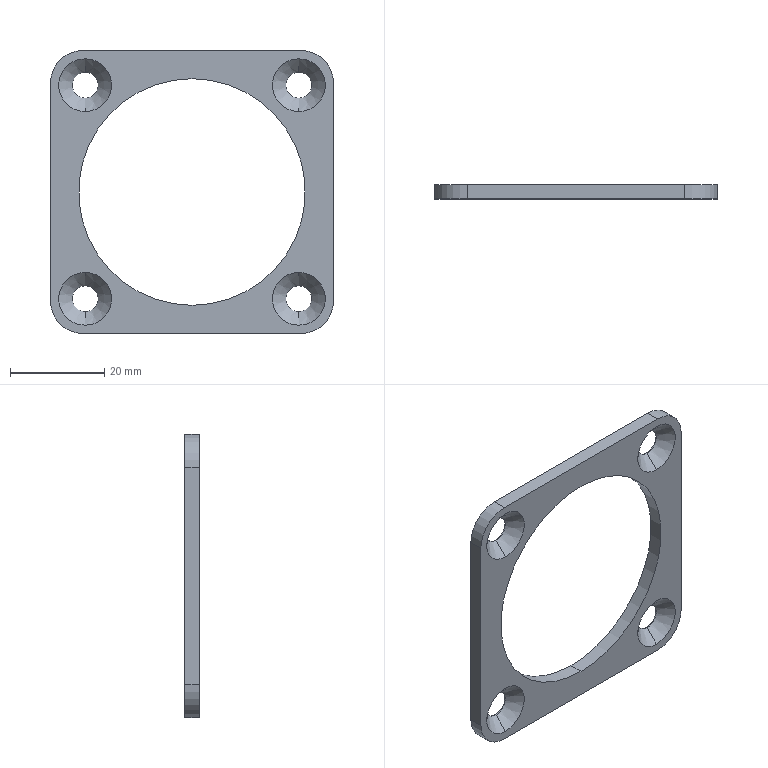Component | SolidWorks | H2020022-0406-1-2 | 1 solid | 28 faces | box 60 x 3 x 60 mm | volume 4582 mm3 | cylinder 14 | cone 8 | plane 6 | commonest cylinder face diameters 5.5 x8 14 x4 48 x2 | material SUS304
build123d program:
from build123d import *

# Parameters (mm, degrees)
SKETCH2_W           = 60
SKETCH2_H           = 60
SKETCH2_R           = 24
BOSS_EXTRUDE1_DEPTH = 3
CIRPATTERN1_COUNT   = 4
FILLET1_R           = 7


with BuildPart() as part:
    # Sketch2 → Boss-Extrude1 (new body)
    with BuildSketch(Plane(origin=(0, 0, 0), x_dir=(1, 0, 0), z_dir=(0, 1, 0))):
        Rectangle(SKETCH2_W, SKETCH2_H)
        with Locations(Location((0, 0, 0), (0, 0, 270))):
            Circle(SKETCH2_R, mode=Mode.SUBTRACT)
    extrude(amount=BOSS_EXTRUDE1_DEPTH)

    # Sketch4 → Countersunk Hole for M5 Hexagon Socket C (revolve, cut)
    with BuildSketch(Plane(origin=(-22.627, 3, -22.627), x_dir=(0, 0, 1), z_dir=(1, 0, 0))):
        Polygon((0, 0), (0, 3), (2.75, 3), (2.75, 2.85), (5.6, 0), align=None)
    countersunk_hole_for_m5_hexagon_socket_c = revolve(axis=Axis((-22.627, 9.35, -22.627), (0, -1, 0)), mode=Mode.SUBTRACT)

    # CirPattern1: Countersunk Hole for M5 Hexagon Socket C ×4 about axis
    cirpattern1_axis = Axis((0, 0, 0), (0, 1, 0))
    for i in range(1, CIRPATTERN1_COUNT):
        add(countersunk_hole_for_m5_hexagon_socket_c.rotate(cirpattern1_axis, i * 360 / CIRPATTERN1_COUNT), mode=Mode.SUBTRACT)

    # Fillet1
    fillet1_edges = [part.edges().sort_by_distance(p)[0] for p in [
        (30, 1.5, 30),
        (-30, 1.5, 30),
        (-30, 1.5, -30),
        (30, 1.5, -30),
    ]]
    fillet(fillet1_edges, radius=FILLET1_R)


solid = part.part

# Placed as in the assembly
solid = solid.moved(Location((-30.964, 101.813, 280.197), (180, 0, 0)))
STEP:
#1=COLOUR_RGB('',0.7922,0.8196,0.9333);
#2=FILL_AREA_STYLE_COLOUR('',#1);
#3=FILL_AREA_STYLE('',(#2));
#4=SURFACE_STYLE_FILL_AREA(#3);
#5=SURFACE_SIDE_STYLE('',(#4));
#6=SURFACE_STYLE_USAGE(.BOTH.,#5);
#7=PRESENTATION_STYLE_ASSIGNMENT((#6));
#8=CARTESIAN_POINT('',(-2.11,4.002,10.032));
#9=VERTEX_POINT('',#8);
#10=CARTESIAN_POINT('',(-2.11,4.002,10.249));
#11=VERTEX_POINT('',#10);
#12=CARTESIAN_POINT('',(-2.11,4.002,10.141));
#13=DIRECTION('',(0.,-1.,0.));
#14=DIRECTION('',(0.,0.,1.));
#15=AXIS2_PLACEMENT_3D('',#12,#13,#14);
#16=CIRCLE('',#15,0.1083);
#17=EDGE_CURVE('',#9,#11,#16,.T.);
#18=ORIENTED_EDGE('',*,*,#17,.F.);
#19=CARTESIAN_POINT('',(-2.11,3.89,9.92));
#20=VERTEX_POINT('',#19);
#21=CARTESIAN_POINT('',(-2.11,3.89,9.92));
#22=DIRECTION('',(-0.,-0.7071,-0.7071));
#23=VECTOR('',#22,39.37);
#24=LINE('',#21,#23);
#25=EDGE_CURVE('',#9,#20,#24,.T.);
#26=ORIENTED_EDGE('',*,*,#25,.T.);
#27=CARTESIAN_POINT('',(-2.11,3.89,10.361));
#28=VERTEX_POINT('',#27);
#29=CARTESIAN_POINT('',(-2.11,3.89,10.141));
#30=DIRECTION('',(0.,-1.,0.));
#31=DIRECTION('',(0.,0.,1.));
#32=AXIS2_PLACEMENT_3D('',#29,#30,#31);
#33=CIRCLE('',#32,0.2205);
#34=EDGE_CURVE('',#20,#28,#33,.T.);
#35=ORIENTED_EDGE('',*,*,#34,.T.);
#36=CARTESIAN_POINT('',(-2.11,3.89,10.361));
#37=DIRECTION('',(0.,-0.7071,0.7071));
#38=VECTOR('',#37,39.37);
#39=LINE('',#36,#38);
#40=EDGE_CURVE('',#11,#28,#39,.T.);
#41=ORIENTED_EDGE('',*,*,#40,.F.);
#42=EDGE_LOOP('',(#18,#26,#35,#41));
#43=FACE_OUTER_BOUND('',#42,.T.);
#44=CARTESIAN_POINT('',(-2.11,3.89,10.141));
#45=DIRECTION('',(0.,-1.,0.));
#46=DIRECTION('',(0.,0.,1.));
#47=AXIS2_PLACEMENT_3D('',#44,#45,#46);
#48=CONICAL_SURFACE('',#47,0.2205,0.7854);
#49=ADVANCED_FACE('',(#43),#48,.F.);
#50=CARTESIAN_POINT('',(-2.11,4.008,10.032));
#51=VERTEX_POINT('',#50);
#52=CARTESIAN_POINT('',(-2.11,4.008,10.249));
#53=VERTEX_POINT('',#52);
#54=CARTESIAN_POINT('',(-2.11,4.008,10.141));
#55=DIRECTION('',(0.,-1.,0.));
#56=DIRECTION('',(0.,0.,1.));
#57=AXIS2_PLACEMENT_3D('',#54,#55,#56);
#58=CIRCLE('',#57,0.1083);
#59=EDGE_CURVE('',#51,#53,#58,.T.);
#60=ORIENTED_EDGE('',*,*,#59,.F.);
#61=CARTESIAN_POINT('',(-2.11,3.89,10.032));
#62=DIRECTION('',(0.,-1.,0.));
#63=VECTOR('',#62,39.37);
#64=LINE('',#61,#63);
#65=EDGE_CURVE('',#51,#9,#64,.T.);
#66=ORIENTED_EDGE('',*,*,#65,.T.);
#67=ORIENTED_EDGE('',*,*,#17,.T.);
#68=CARTESIAN_POINT('',(-2.11,3.89,10.249));
#69=DIRECTION('',(0.,-1.,0.));
#70=VECTOR('',#69,39.37);
#71=LINE('',#68,#70);
#72=EDGE_CURVE('',#53,#11,#71,.T.);
#73=ORIENTED_EDGE('',*,*,#72,.F.);
#74=EDGE_LOOP('',(#60,#66,#67,#73));
#75=FACE_OUTER_BOUND('',#74,.T.);
#76=CARTESIAN_POINT('',(-2.11,3.89,10.141));
#77=DIRECTION('',(0.,-1.,0.));
#78=DIRECTION('',(0.,0.,1.));
#79=AXIS2_PLACEMENT_3D('',#76,#77,#78);
#80=CYLINDRICAL_SURFACE('',#79,0.1083);
#81=ADVANCED_FACE('',(#75),#80,.F.);
#82=CARTESIAN_POINT('',(-2.11,4.002,11.814));
#83=VERTEX_POINT('',#82);
#84=CARTESIAN_POINT('',(-2.11,4.002,12.03));
#85=VERTEX_POINT('',#84);
#86=CARTESIAN_POINT('',(-2.11,4.002,11.922));
#87=DIRECTION('',(0.,-1.,0.));
#88=DIRECTION('',(0.,0.,1.));
#89=AXIS2_PLACEMENT_3D('',#86,#87,#88);
#90=CIRCLE('',#89,0.1083);
#91=EDGE_CURVE('',#83,#85,#90,.T.);
#92=ORIENTED_EDGE('',*,*,#91,.F.);
#93=CARTESIAN_POINT('',(-2.11,3.89,11.702));
#94=VERTEX_POINT('',#93);
#95=CARTESIAN_POINT('',(-2.11,3.89,11.702));
#96=DIRECTION('',(-0.,-0.7071,-0.7071));
#97=VECTOR('',#96,39.37);
#98=LINE('',#95,#97);
#99=EDGE_CURVE('',#83,#94,#98,.T.);
#100=ORIENTED_EDGE('',*,*,#99,.T.);
#101=CARTESIAN_POINT('',(-2.11,3.89,12.143));
#102=VERTEX_POINT('',#101);
#103=CARTESIAN_POINT('',(-2.11,3.89,11.922));
#104=DIRECTION('',(0.,-1.,0.));
#105=DIRECTION('',(0.,0.,1.));
#106=AXIS2_PLACEMENT_3D('',#103,#104,#105);
#107=CIRCLE('',#106,0.2205);
#108=EDGE_CURVE('',#94,#102,#107,.T.);
#109=ORIENTED_EDGE('',*,*,#108,.T.);
#110=CARTESIAN_POINT('',(-2.11,3.89,12.143));
#111=DIRECTION('',(0.,-0.7071,0.7071));
#112=VECTOR('',#111,39.37);
#113=LINE('',#110,#112);
#114=EDGE_CURVE('',#85,#102,#113,.T.);
#115=ORIENTED_EDGE('',*,*,#114,.F.);
#116=EDGE_LOOP('',(#92,#100,#109,#115));
#117=FACE_OUTER_BOUND('',#116,.T.);
#118=CARTESIAN_POINT('',(-2.11,3.89,11.922));
#119=DIRECTION('',(0.,-1.,0.));
#120=DIRECTION('',(0.,0.,1.));
#121=AXIS2_PLACEMENT_3D('',#118,#119,#120);
#122=CONICAL_SURFACE('',#121,0.2205,0.7854);
#123=ADVANCED_FACE('',(#117),#122,.F.);
#124=CARTESIAN_POINT('',(-2.11,4.008,11.814));
#125=VERTEX_POINT('',#124);
#126=CARTESIAN_POINT('',(-2.11,4.008,12.03));
#127=VERTEX_POINT('',#126);
#128=CARTESIAN_POINT('',(-2.11,4.008,11.922));
#129=DIRECTION('',(0.,-1.,0.));
#130=DIRECTION('',(0.,0.,1.));
#131=AXIS2_PLACEMENT_3D('',#128,#129,#130);
#132=CIRCLE('',#131,0.1083);
#133=EDGE_CURVE('',#125,#127,#132,.T.);
#134=ORIENTED_EDGE('',*,*,#133,.F.);
#135=CARTESIAN_POINT('',(-2.11,3.89,11.814));
#136=DIRECTION('',(0.,-1.,0.));
#137=VECTOR('',#136,39.37);
#138=LINE('',#135,#137);
#139=EDGE_CURVE('',#125,#83,#138,.T.);
#140=ORIENTED_EDGE('',*,*,#139,.T.);
#141=ORIENTED_EDGE('',*,*,#91,.T.);
#142=CARTESIAN_POINT('',(-2.11,3.89,12.03));
#143=DIRECTION('',(0.,-1.,0.));
#144=VECTOR('',#143,39.37);
#145=LINE('',#142,#144);
#146=EDGE_CURVE('',#127,#85,#145,.T.);
#147=ORIENTED_EDGE('',*,*,#146,.F.);
#148=EDGE_LOOP('',(#134,#140,#141,#147));
#149=FACE_OUTER_BOUND('',#148,.T.);
#150=CARTESIAN_POINT('',(-2.11,3.89,11.922));
#151=DIRECTION('',(0.,-1.,0.));
#152=DIRECTION('',(0.,0.,1.));
#153=AXIS2_PLACEMENT_3D('',#150,#151,#152);
#154=CYLINDRICAL_SURFACE('',#153,0.1083);
#155=ADVANCED_FACE('',(#149),#154,.F.);
#156=CARTESIAN_POINT('',(-0.3282,4.002,11.814));
#157=VERTEX_POINT('',#156);
#158=CARTESIAN_POINT('',(-0.3282,4.002,12.03));
#159=VERTEX_POINT('',#158);
#160=CARTESIAN_POINT('',(-0.3282,4.002,11.922));
#161=DIRECTION('',(0.,-1.,0.));
#162=DIRECTION('',(0.,0.,1.));
#163=AXIS2_PLACEMENT_3D('',#160,#161,#162);
#164=CIRCLE('',#163,0.1083);
#165=EDGE_CURVE('',#157,#159,#164,.T.);
#166=ORIENTED_EDGE('',*,*,#165,.F.);
#167=CARTESIAN_POINT('',(-0.3282,3.89,11.702));
#168=VERTEX_POINT('',#167);
#169=CARTESIAN_POINT('',(-0.3282,3.89,11.702));
#170=DIRECTION('',(-0.,-0.7071,-0.7071));
#171=VECTOR('',#170,39.37);
#172=LINE('',#169,#171);
#173=EDGE_CURVE('',#157,#168,#172,.T.);
#174=ORIENTED_EDGE('',*,*,#173,.T.);
#175=CARTESIAN_POINT('',(-0.3282,3.89,12.143));
#176=VERTEX_POINT('',#175);
#177=CARTESIAN_POINT('',(-0.3282,3.89,11.922));
#178=DIRECTION('',(0.,-1.,0.));
#179=DIRECTION('',(0.,0.,1.));
#180=AXIS2_PLACEMENT_3D('',#177,#178,#179);
#181=CIRCLE('',#180,0.2205);
#182=EDGE_CURVE('',#168,#176,#181,.T.);
#183=ORIENTED_EDGE('',*,*,#182,.T.);
#184=CARTESIAN_POINT('',(-0.3282,3.89,12.143));
#185=DIRECTION('',(0.,-0.7071,0.7071));
#186=VECTOR('',#185,39.37);
#187=LINE('',#184,#186);
#188=EDGE_CURVE('',#159,#176,#187,.T.);
#189=ORIENTED_EDGE('',*,*,#188,.F.);
#190=EDGE_LOOP('',(#166,#174,#183,#189));
#191=FACE_OUTER_BOUND('',#190,.T.);
#192=CARTESIAN_POINT('',(-0.3282,3.89,11.922));
#193=DIRECTION('',(0.,-1.,0.));
#194=DIRECTION('',(0.,0.,1.));
#195=AXIS2_PLACEMENT_3D('',#192,#193,#194);
#196=CONICAL_SURFACE('',#195,0.2205,0.7854);
#197=ADVANCED_FACE('',(#191),#196,.F.);
#198=CARTESIAN_POINT('',(-0.3282,4.008,11.814));
#199=VERTEX_POINT('',#198);
#200=CARTESIAN_POINT('',(-0.3282,4.008,12.03));
#201=VERTEX_POINT('',#200);
#202=CARTESIAN_POINT('',(-0.3282,4.008,11.922));
#203=DIRECTION('',(0.,-1.,0.));
#204=DIRECTION('',(0.,0.,1.));
#205=AXIS2_PLACEMENT_3D('',#202,#203,#204);
#206=CIRCLE('',#205,0.1083);
#207=EDGE_CURVE('',#199,#201,#206,.T.);
#208=ORIENTED_EDGE('',*,*,#207,.F.);
#209=CARTESIAN_POINT('',(-0.3282,3.89,11.814));
#210=DIRECTION('',(0.,-1.,0.));
#211=VECTOR('',#210,39.37);
#212=LINE('',#209,#211);
#213=EDGE_CURVE('',#199,#157,#212,.T.);
#214=ORIENTED_EDGE('',*,*,#213,.T.);
#215=ORIENTED_EDGE('',*,*,#165,.T.);
#216=CARTESIAN_POINT('',(-0.3282,3.89,12.03));
#217=DIRECTION('',(0.,-1.,0.));
#218=VECTOR('',#217,39.37);
#219=LINE('',#216,#218);
#220=EDGE_CURVE('',#201,#159,#219,.T.);
#221=ORIENTED_EDGE('',*,*,#220,.F.);
#222=EDGE_LOOP('',(#208,#214,#215,#221));
#223=FACE_OUTER_BOUND('',#222,.T.);
#224=CARTESIAN_POINT('',(-0.3282,3.89,11.922));
#225=DIRECTION('',(0.,-1.,0.));
#226=DIRECTION('',(0.,0.,1.));
#227=AXIS2_PLACEMENT_3D('',#224,#225,#226);
#228=CYLINDRICAL_SURFACE('',#227,0.1083);
#229=ADVANCED_FACE('',(#223),#228,.F.);
#230=CARTESIAN_POINT('',(-0.3282,4.002,10.032));
#231=VERTEX_POINT('',#230);
#232=CARTESIAN_POINT('',(-0.3282,4.002,10.249));
#233=VERTEX_POINT('',#232);
#234=CARTESIAN_POINT('',(-0.3282,4.002,10.141));
#235=DIRECTION('',(0.,-1.,0.));
#236=DIRECTION('',(0.,0.,1.));
#237=AXIS2_PLACEMENT_3D('',#234,#235,#236);
#238=CIRCLE('',#237,0.1083);
#239=EDGE_CURVE('',#231,#233,#238,.T.);
#240=ORIENTED_EDGE('',*,*,#239,.F.);
#241=CARTESIAN_POINT('',(-0.3282,3.89,9.92));
#242=VERTEX_POINT('',#241);
#243=CARTESIAN_POINT('',(-0.3282,3.89,9.92));
#244=DIRECTION('',(-0.,-0.7071,-0.7071));
#245=VECTOR('',#244,39.37);
#246=LINE('',#243,#245);
#247=EDGE_CURVE('',#231,#242,#246,.T.);
#248=ORIENTED_EDGE('',*,*,#247,.T.);
#249=CARTESIAN_POINT('',(-0.3282,3.89,10.361));
#250=VERTEX_POINT('',#249);
#251=CARTESIAN_POINT('',(-0.3282,3.89,10.141));
#252=DIRECTION('',(0.,-1.,0.));
#253=DIRECTION('',(0.,0.,1.));
#254=AXIS2_PLACEMENT_3D('',#251,#252,#253);
#255=CIRCLE('',#254,0.2205);
#256=EDGE_CURVE('',#242,#250,#255,.T.);
#257=ORIENTED_EDGE('',*,*,#256,.T.);
#258=CARTESIAN_POINT('',(-0.3282,3.89,10.361));
#259=DIRECTION('',(0.,-0.7071,0.7071));
#260=VECTOR('',#259,39.37);
#261=LINE('',#258,#260);
#262=EDGE_CURVE('',#233,#250,#261,.T.);
#263=ORIENTED_EDGE('',*,*,#262,.F.);
#264=EDGE_LOOP('',(#240,#248,#257,#263));
#265=FACE_OUTER_BOUND('',#264,.T.);
#266=CARTESIAN_POINT('',(-0.3282,3.89,10.141));
#267=DIRECTION('',(0.,-1.,0.));
#268=DIRECTION('',(0.,0.,1.));
#269=AXIS2_PLACEMENT_3D('',#266,#267,#268);
#270=CONICAL_SURFACE('',#269,0.2205,0.7854);
#271=ADVANCED_FACE('',(#265),#270,.F.);
#272=CARTESIAN_POINT('',(-0.3282,4.008,10.032));
#273=VERTEX_POINT('',#272);
#274=CARTESIAN_POINT('',(-0.3282,4.008,10.249));
#275=VERTEX_POINT('',#274);
#276=CARTESIAN_POINT('',(-0.3282,4.008,10.141));
#277=DIRECTION('',(0.,-1.,0.));
#278=DIRECTION('',(0.,0.,1.));
#279=AXIS2_PLACEMENT_3D('',#276,#277,#278);
#280=CIRCLE('',#279,0.1083);
#281=EDGE_CURVE('',#273,#275,#280,.T.);
#282=ORIENTED_EDGE('',*,*,#281,.F.);
#283=CARTESIAN_POINT('',(-0.3282,3.89,10.032));
#284=DIRECTION('',(0.,-1.,0.));
#285=VECTOR('',#284,39.37);
#286=LINE('',#283,#285);
#287=EDGE_CURVE('',#273,#231,#286,.T.);
#288=ORIENTED_EDGE('',*,*,#287,.T.);
#289=ORIENTED_EDGE('',*,*,#239,.T.);
#290=CARTESIAN_POINT('',(-0.3282,3.89,10.249));
#291=DIRECTION('',(0.,-1.,0.));
#292=VECTOR('',#291,39.37);
#293=LINE('',#290,#292);
#294=EDGE_CURVE('',#275,#233,#293,.T.);
#295=ORIENTED_EDGE('',*,*,#294,.F.);
#296=EDGE_LOOP('',(#282,#288,#289,#295));
#297=FACE_OUTER_BOUND('',#296,.T.);
#298=CARTESIAN_POINT('',(-0.3282,3.89,10.141));
#299=DIRECTION('',(0.,-1.,0.));
#300=DIRECTION('',(0.,0.,1.));
#301=AXIS2_PLACEMENT_3D('',#298,#299,#300);
#302=CYLINDRICAL_SURFACE('',#301,0.1083);
#303=ADVANCED_FACE('',(#297),#302,.F.);
#304=CARTESIAN_POINT('',(-1.219,3.89,10.086));
#305=VERTEX_POINT('',#304);
#306=CARTESIAN_POINT('',(-1.219,3.89,11.976));
#307=VERTEX_POINT('',#306);
#308=CARTESIAN_POINT('',(-1.219,3.89,11.031));
#309=DIRECTION('',(0.,-1.,0.));
#310=DIRECTION('',(0.,0.,1.));
#311=AXIS2_PLACEMENT_3D('',#308,#309,#310);
#312=CIRCLE('',#311,0.9449);
#313=EDGE_CURVE('',#305,#307,#312,.T.);
#314=ORIENTED_EDGE('',*,*,#313,.T.);
#315=CARTESIAN_POINT('',(-1.219,4.008,11.976));
#316=VERTEX_POINT('',#315);
#317=CARTESIAN_POINT('',(-1.219,3.89,11.976));
#318=DIRECTION('',(0.,1.,0.));
#319=VECTOR('',#318,39.37);
#320=LINE('',#317,#319);
#321=EDGE_CURVE('',#307,#316,#320,.T.);
#322=ORIENTED_EDGE('',*,*,#321,.T.);
#323=CARTESIAN_POINT('',(-1.219,4.008,10.086));
#324=VERTEX_POINT('',#323);
#325=CARTESIAN_POINT('',(-1.219,4.008,11.031));
#326=DIRECTION('',(0.,-1.,0.));
#327=DIRECTION('',(0.,0.,1.));
#328=AXIS2_PLACEMENT_3D('',#325,#326,#327);
#329=CIRCLE('',#328,0.9449);
#330=EDGE_CURVE('',#324,#316,#329,.T.);
#331=ORIENTED_EDGE('',*,*,#330,.F.);
#332=CARTESIAN_POINT('',(-1.219,3.89,10.086));
#333=DIRECTION('',(0.,1.,0.));
#334=VECTOR('',#333,39.37);
#335=LINE('',#332,#334);
#336=EDGE_CURVE('',#305,#324,#335,.T.);
#337=ORIENTED_EDGE('',*,*,#336,.F.);
#338=EDGE_LOOP('',(#314,#322,#331,#337));
#339=FACE_OUTER_BOUND('',#338,.T.);
#340=CARTESIAN_POINT('',(-1.219,3.89,11.031));
#341=DIRECTION('',(0.,1.,0.));
#342=DIRECTION('',(-0.,0.,-1.));
#343=AXIS2_PLACEMENT_3D('',#340,#341,#342);
#344=CYLINDRICAL_SURFACE('',#343,0.9449);
#345=ADVANCED_FACE('',(#339),#344,.F.);
#346=CARTESIAN_POINT('',(-2.11,3.89,10.141));
#347=DIRECTION('',(0.,-1.,0.));
#348=DIRECTION('',(0.,0.,1.));
#349=AXIS2_PLACEMENT_3D('',#346,#347,#348);
#350=CIRCLE('',#349,0.2205);
#351=EDGE_CURVE('',#28,#20,#350,.T.);
#352=ORIENTED_EDGE('',*,*,#351,.F.);
#353=ORIENTED_EDGE('',*,*,#34,.F.);
#354=EDGE_LOOP('',(#352,#353));
#355=FACE_BOUND('',#354,.T.);
#356=CARTESIAN_POINT('',(-2.11,3.89,11.922));
#357=DIRECTION('',(0.,-1.,0.));
#358=DIRECTION('',(0.,0.,1.));
#359=AXIS2_PLACEMENT_3D('',#356,#357,#358);
#360=CIRCLE('',#359,0.2205);
#361=EDGE_CURVE('',#102,#94,#360,.T.);
#362=ORIENTED_EDGE('',*,*,#361,.F.);
#363=ORIENTED_EDGE('',*,*,#108,.F.);
#364=EDGE_LOOP('',(#362,#363));
#365=FACE_BOUND('',#364,.T.);
#366=CARTESIAN_POINT('',(-0.3282,3.89,11.922));
#367=DIRECTION('',(0.,-1.,0.));
#368=DIRECTION('',(0.,0.,1.));
#369=AXIS2_PLACEMENT_3D('',#366,#367,#368);
#370=CIRCLE('',#369,0.2205);
#371=EDGE_CURVE('',#176,#168,#370,.T.);
#372=ORIENTED_EDGE('',*,*,#371,.F.);
#373=ORIENTED_EDGE('',*,*,#182,.F.);
#374=EDGE_LOOP('',(#372,#373));
#375=FACE_BOUND('',#374,.T.);
#376=CARTESIAN_POINT('',(-0.3282,3.89,10.141));
#377=DIRECTION('',(0.,-1.,0.));
#378=DIRECTION('',(0.,0.,1.));
#379=AXIS2_PLACEMENT_3D('',#376,#377,#378);
#380=CIRCLE('',#379,0.2205);
#381=EDGE_CURVE('',#250,#242,#380,.T.);
#382=ORIENTED_EDGE('',*,*,#381,.F.);
#383=ORIENTED_EDGE('',*,*,#256,.F.);
#384=EDGE_LOOP('',(#382,#383));
#385=FACE_BOUND('',#384,.T.);
#386=CARTESIAN_POINT('',(-0.03796,3.89,10.126));
#387=VERTEX_POINT('',#386);
#388=CARTESIAN_POINT('',(-0.03796,3.89,11.937));
#389=VERTEX_POINT('',#388);
#390=CARTESIAN_POINT('',(-0.03796,3.89,9.85));
#391=DIRECTION('',(0.,0.,1.));
#392=VECTOR('',#391,39.37);
#393=LINE('',#390,#392);
#394=EDGE_CURVE('',#387,#389,#393,.T.);
#395=ORIENTED_EDGE('',*,*,#394,.T.);
#396=CARTESIAN_POINT('',(-0.3136,3.89,12.212));
#397=VERTEX_POINT('',#396);
#398=CARTESIAN_POINT('',(-0.3136,3.89,11.937));
#399=DIRECTION('',(0.,-1.,0.));
#400=DIRECTION('',(0.,0.,1.));
#401=AXIS2_PLACEMENT_3D('',#398,#399,#400);
#402=CIRCLE('',#401,0.2756);
#403=EDGE_CURVE('',#389,#397,#402,.T.);
#404=ORIENTED_EDGE('',*,*,#403,.T.);
#405=CARTESIAN_POINT('',(-2.125,3.89,12.212));
#406=VERTEX_POINT('',#405);
#407=CARTESIAN_POINT('',(-0.03796,3.89,12.212));
#408=DIRECTION('',(-1.,0.,0.));
#409=VECTOR('',#408,39.37);
#410=LINE('',#407,#409);
#411=EDGE_CURVE('',#397,#406,#410,.T.);
#412=ORIENTED_EDGE('',*,*,#411,.T.);
#413=CARTESIAN_POINT('',(-2.4,3.89,11.937));
#414=VERTEX_POINT('',#413);
#415=CARTESIAN_POINT('',(-2.125,3.89,11.937));
#416=DIRECTION('',(0.,-1.,0.));
#417=DIRECTION('',(0.,0.,1.));
#418=AXIS2_PLACEMENT_3D('',#415,#416,#417);
#419=CIRCLE('',#418,0.2756);
#420=EDGE_CURVE('',#406,#414,#419,.T.);
#421=ORIENTED_EDGE('',*,*,#420,.T.);
#422=CARTESIAN_POINT('',(-2.4,3.89,10.126));
#423=VERTEX_POINT('',#422);
#424=CARTESIAN_POINT('',(-2.4,3.89,9.85));
#425=DIRECTION('',(-0.,0.,-1.));
#426=VECTOR('',#425,39.37);
#427=LINE('',#424,#426);
#428=EDGE_CURVE('',#414,#423,#427,.T.);
#429=ORIENTED_EDGE('',*,*,#428,.T.);
#430=CARTESIAN_POINT('',(-2.125,3.89,9.85));
#431=VERTEX_POINT('',#430);
#432=CARTESIAN_POINT('',(-2.125,3.89,10.126));
#433=DIRECTION('',(0.,-1.,0.));
#434=DIRECTION('',(0.,0.,1.));
#435=AXIS2_PLACEMENT_3D('',#432,#433,#434);
#436=CIRCLE('',#435,0.2756);
#437=EDGE_CURVE('',#423,#431,#436,.T.);
#438=ORIENTED_EDGE('',*,*,#437,.T.);
#439=CARTESIAN_POINT('',(-0.3136,3.89,9.85));
#440=VERTEX_POINT('',#439);
#441=CARTESIAN_POINT('',(-0.03796,3.89,9.85));
#442=DIRECTION('',(1.,0.,-0.));
#443=VECTOR('',#442,39.37);
#444=LINE('',#441,#443);
#445=EDGE_CURVE('',#431,#440,#444,.T.);
#446=ORIENTED_EDGE('',*,*,#445,.T.);
#447=CARTESIAN_POINT('',(-0.3136,3.89,10.126));
#448=DIRECTION('',(0.,-1.,0.));
#449=DIRECTION('',(0.,0.,1.));
#450=AXIS2_PLACEMENT_3D('',#447,#448,#449);
#451=CIRCLE('',#450,0.2756);
#452=EDGE_CURVE('',#440,#387,#451,.T.);
#453=ORIENTED_EDGE('',*,*,#452,.T.);
#454=EDGE_LOOP('',(#395,#404,#412,#421,#429,#438,#446,#453));
#455=FACE_OUTER_BOUND('',#454,.T.);
#456=ORIENTED_EDGE('',*,*,#313,.F.);
#457=CARTESIAN_POINT('',(-1.219,3.89,11.031));
#458=DIRECTION('',(0.,-1.,0.));
#459=DIRECTION('',(0.,0.,1.));
#460=AXIS2_PLACEMENT_3D('',#457,#458,#459);
#461=CIRCLE('',#460,0.9449);
#462=EDGE_CURVE('',#307,#305,#461,.T.);
#463=ORIENTED_EDGE('',*,*,#462,.F.);
#464=EDGE_LOOP('',(#456,#463));
#465=FACE_BOUND('',#464,.T.);
#466=CARTESIAN_POINT('',(-1.219,3.89,11.031));
#467=DIRECTION('',(0.,-1.,0.));
#468=DIRECTION('',(0.,0.,1.));
#469=AXIS2_PLACEMENT_3D('',#466,#467,#468);
#470=PLANE('',#469);
#471=ADVANCED_FACE('',(#355,#365,#375,#385,#455,#465),#470,.T.);
#472=CARTESIAN_POINT('',(-2.11,4.008,10.141));
#473=DIRECTION('',(0.,-1.,0.));
#474=DIRECTION('',(0.,0.,1.));
#475=AXIS2_PLACEMENT_3D('',#472,#473,#474);
#476=CIRCLE('',#475,0.1083);
#477=EDGE_CURVE('',#53,#51,#476,.T.);
#478=ORIENTED_EDGE('',*,*,#477,.T.);
#479=ORIENTED_EDGE('',*,*,#59,.T.);
#480=EDGE_LOOP('',(#478,#479));
#481=FACE_BOUND('',#480,.T.);
#482=CARTESIAN_POINT('',(-2.11,4.008,11.922));
#483=DIRECTION('',(0.,-1.,0.));
#484=DIRECTION('',(0.,0.,1.));
#485=AXIS2_PLACEMENT_3D('',#482,#483,#484);
#486=CIRCLE('',#485,0.1083);
#487=EDGE_CURVE('',#127,#125,#486,.T.);
#488=ORIENTED_EDGE('',*,*,#487,.T.);
#489=ORIENTED_EDGE('',*,*,#133,.T.);
#490=EDGE_LOOP('',(#488,#489));
#491=FACE_BOUND('',#490,.T.);
#492=CARTESIAN_POINT('',(-0.3282,4.008,11.922));
#493=DIRECTION('',(0.,-1.,0.));
#494=DIRECTION('',(0.,0.,1.));
#495=AXIS2_PLACEMENT_3D('',#492,#493,#494);
#496=CIRCLE('',#495,0.1083);
#497=EDGE_CURVE('',#201,#199,#496,.T.);
#498=ORIENTED_EDGE('',*,*,#497,.T.);
#499=ORIENTED_EDGE('',*,*,#207,.T.);
#500=EDGE_LOOP('',(#498,#499));
#501=FACE_BOUND('',#500,.T.);
#502=CARTESIAN_POINT('',(-0.3282,4.008,10.141));
#503=DIRECTION('',(0.,-1.,0.));
#504=DIRECTION('',(0.,0.,1.));
#505=AXIS2_PLACEMENT_3D('',#502,#503,#504);
#506=CIRCLE('',#505,0.1083);
#507=EDGE_CURVE('',#275,#273,#506,.T.);
#508=ORIENTED_EDGE('',*,*,#507,.T.);
#509=ORIENTED_EDGE('',*,*,#281,.T.);
#510=EDGE_LOOP('',(#508,#509));
#511=FACE_BOUND('',#510,.T.);
#512=CARTESIAN_POINT('',(-0.3136,4.008,12.212));
#513=VERTEX_POINT('',#512);
#514=CARTESIAN_POINT('',(-2.125,4.008,12.212));
#515=VERTEX_POINT('',#514);
#516=CARTESIAN_POINT('',(-0.03796,4.008,12.212));
#517=DIRECTION('',(-1.,0.,0.));
#518=VECTOR('',#517,39.37);
#519=LINE('',#516,#518);
#520=EDGE_CURVE('',#513,#515,#519,.T.);
#521=ORIENTED_EDGE('',*,*,#520,.F.);
#522=CARTESIAN_POINT('',(-0.03796,4.008,11.937));
#523=VERTEX_POINT('',#522);
#524=CARTESIAN_POINT('',(-0.3136,4.008,11.937));
#525=DIRECTION('',(0.,1.,0.));
#526=DIRECTION('',(0.,0.,1.));
#527=AXIS2_PLACEMENT_3D('',#524,#525,#526);
#528=CIRCLE('',#527,0.2756);
#529=EDGE_CURVE('',#513,#523,#528,.T.);
#530=ORIENTED_EDGE('',*,*,#529,.T.);
#531=CARTESIAN_POINT('',(-0.03796,4.008,10.126));
#532=VERTEX_POINT('',#531);
#533=CARTESIAN_POINT('',(-0.03796,4.008,9.85));
#534=DIRECTION('',(0.,0.,1.));
#535=VECTOR('',#534,39.37);
#536=LINE('',#533,#535);
#537=EDGE_CURVE('',#532,#523,#536,.T.);
#538=ORIENTED_EDGE('',*,*,#537,.F.);
#539=CARTESIAN_POINT('',(-0.3136,4.008,9.85));
#540=VERTEX_POINT('',#539);
#541=CARTESIAN_POINT('',(-0.3136,4.008,10.126));
#542=DIRECTION('',(0.,1.,0.));
#543=DIRECTION('',(0.,0.,1.));
#544=AXIS2_PLACEMENT_3D('',#541,#542,#543);
#545=CIRCLE('',#544,0.2756);
#546=EDGE_CURVE('',#532,#540,#545,.T.);
#547=ORIENTED_EDGE('',*,*,#546,.T.);
#548=CARTESIAN_POINT('',(-2.125,4.008,9.85));
#549=VERTEX_POINT('',#548);
#550=CARTESIAN_POINT('',(-0.03796,4.008,9.85));
#551=DIRECTION('',(1.,0.,-0.));
#552=VECTOR('',#551,39.37);
#553=LINE('',#550,#552);
#554=EDGE_CURVE('',#549,#540,#553,.T.);
#555=ORIENTED_EDGE('',*,*,#554,.F.);
#556=CARTESIAN_POINT('',(-2.4,4.008,10.126));
#557=VERTEX_POINT('',#556);
#558=CARTESIAN_POINT('',(-2.125,4.008,10.126));
#559=DIRECTION('',(0.,1.,0.));
#560=DIRECTION('',(0.,0.,1.));
#561=AXIS2_PLACEMENT_3D('',#558,#559,#560);
#562=CIRCLE('',#561,0.2756);
#563=EDGE_CURVE('',#549,#557,#562,.T.);
#564=ORIENTED_EDGE('',*,*,#563,.T.);
#565=CARTESIAN_POINT('',(-2.4,4.008,11.937));
#566=VERTEX_POINT('',#565);
#567=CARTESIAN_POINT('',(-2.4,4.008,9.85));
#568=DIRECTION('',(-0.,0.,-1.));
#569=VECTOR('',#568,39.37);
#570=LINE('',#567,#569);
#571=EDGE_CURVE('',#566,#557,#570,.T.);
#572=ORIENTED_EDGE('',*,*,#571,.F.);
#573=CARTESIAN_POINT('',(-2.125,4.008,11.937));
#574=DIRECTION('',(0.,1.,0.));
#575=DIRECTION('',(0.,0.,1.));
#576=AXIS2_PLACEMENT_3D('',#573,#574,#575);
#577=CIRCLE('',#576,0.2756);
#578=EDGE_CURVE('',#566,#515,#577,.T.);
#579=ORIENTED_EDGE('',*,*,#578,.T.);
#580=EDGE_LOOP('',(#521,#530,#538,#547,#555,#564,#572,#579));
#581=FACE_OUTER_BOUND('',#580,.T.);
#582=ORIENTED_EDGE('',*,*,#330,.T.);
#583=CARTESIAN_POINT('',(-1.219,4.008,11.031));
#584=DIRECTION('',(0.,-1.,0.));
#585=DIRECTION('',(0.,0.,1.));
#586=AXIS2_PLACEMENT_3D('',#583,#584,#585);
#587=CIRCLE('',#586,0.9449);
#588=EDGE_CURVE('',#316,#324,#587,.T.);
#589=ORIENTED_EDGE('',*,*,#588,.T.);
#590=EDGE_LOOP('',(#582,#589));
#591=FACE_BOUND('',#590,.T.);
#592=CARTESIAN_POINT('',(-1.219,4.008,11.031));
#593=DIRECTION('',(0.,-1.,0.));
#594=DIRECTION('',(0.,0.,1.));
#595=AXIS2_PLACEMENT_3D('',#592,#593,#594);
#596=PLANE('',#595);
#597=ADVANCED_FACE('',(#481,#491,#501,#511,#581,#591),#596,.F.);
#598=ORIENTED_EDGE('',*,*,#428,.F.);
#599=CARTESIAN_POINT('',(-2.4,3.89,11.937));
#600=DIRECTION('',(0.,1.,0.));
#601=VECTOR('',#600,39.37);
#602=LINE('',#599,#601);
#603=EDGE_CURVE('',#414,#566,#602,.T.);
#604=ORIENTED_EDGE('',*,*,#603,.T.);
#605=ORIENTED_EDGE('',*,*,#571,.T.);
#606=CARTESIAN_POINT('',(-2.4,3.89,10.126));
#607=DIRECTION('',(0.,-1.,0.));
#608=VECTOR('',#607,39.37);
#609=LINE('',#606,#608);
#610=EDGE_CURVE('',#557,#423,#609,.T.);
#611=ORIENTED_EDGE('',*,*,#610,.T.);
#612=EDGE_LOOP('',(#598,#604,#605,#611));
#613=FACE_OUTER_BOUND('',#612,.T.);
#614=CARTESIAN_POINT('',(-2.4,3.89,9.85));
#615=DIRECTION('',(1.,0.,-0.));
#616=DIRECTION('',(0.,0.,1.));
#617=AXIS2_PLACEMENT_3D('',#614,#615,#616);
#618=PLANE('',#617);
#619=ADVANCED_FACE('',(#613),#618,.F.);
#620=ORIENTED_EDGE('',*,*,#445,.F.);
#621=CARTESIAN_POINT('',(-2.125,3.89,9.85));
#622=DIRECTION('',(0.,1.,0.));
#623=VECTOR('',#622,39.37);
#624=LINE('',#621,#623);
#625=EDGE_CURVE('',#431,#549,#624,.T.);
#626=ORIENTED_EDGE('',*,*,#625,.T.);
#627=ORIENTED_EDGE('',*,*,#554,.T.);
#628=CARTESIAN_POINT('',(-0.3136,3.89,9.85));
#629=DIRECTION('',(0.,-1.,0.));
#630=VECTOR('',#629,39.37);
#631=LINE('',#628,#630);
#632=EDGE_CURVE('',#540,#440,#631,.T.);
#633=ORIENTED_EDGE('',*,*,#632,.T.);
#634=EDGE_LOOP('',(#620,#626,#627,#633));
#635=FACE_OUTER_BOUND('',#634,.T.);
#636=CARTESIAN_POINT('',(-0.03796,3.89,9.85));
#637=DIRECTION('',(0.,0.,1.));
#638=DIRECTION('',(-1.,0.,0.));
#639=AXIS2_PLACEMENT_3D('',#636,#637,#638);
#640=PLANE('',#639);
#641=ADVANCED_FACE('',(#635),#640,.F.);
#642=ORIENTED_EDGE('',*,*,#537,.T.);
#643=CARTESIAN_POINT('',(-0.03796,3.89,11.937));
#644=DIRECTION('',(0.,-1.,0.));
#645=VECTOR('',#644,39.37);
#646=LINE('',#643,#645);
#647=EDGE_CURVE('',#523,#389,#646,.T.);
#648=ORIENTED_EDGE('',*,*,#647,.T.);
#649=ORIENTED_EDGE('',*,*,#394,.F.);
#650=CARTESIAN_POINT('',(-0.03796,3.89,10.126));
#651=DIRECTION('',(0.,1.,0.));
#652=VECTOR('',#651,39.37);
#653=LINE('',#650,#652);
#654=EDGE_CURVE('',#387,#532,#653,.T.);
#655=ORIENTED_EDGE('',*,*,#654,.T.);
#656=EDGE_LOOP('',(#642,#648,#649,#655));
#657=FACE_OUTER_BOUND('',#656,.T.);
#658=CARTESIAN_POINT('',(-0.03796,3.89,9.85));
#659=DIRECTION('',(-1.,0.,0.));
#660=DIRECTION('',(-0.,0.,-1.));
#661=AXIS2_PLACEMENT_3D('',#658,#659,#660);
#662=PLANE('',#661);
#663=ADVANCED_FACE('',(#657),#662,.F.);
#664=ORIENTED_EDGE('',*,*,#411,.F.);
#665=CARTESIAN_POINT('',(-0.3136,3.89,12.212));
#666=DIRECTION('',(0.,1.,0.));
#667=VECTOR('',#666,39.37);
#668=LINE('',#665,#667);
#669=EDGE_CURVE('',#397,#513,#668,.T.);
#670=ORIENTED_EDGE('',*,*,#669,.T.);
#671=ORIENTED_EDGE('',*,*,#520,.T.);
#672=CARTESIAN_POINT('',(-2.125,3.89,12.212));
#673=DIRECTION('',(0.,-1.,0.));
#674=VECTOR('',#673,39.37);
#675=LINE('',#672,#674);
#676=EDGE_CURVE('',#515,#406,#675,.T.);
#677=ORIENTED_EDGE('',*,*,#676,.T.);
#678=EDGE_LOOP('',(#664,#670,#671,#677));
#679=FACE_OUTER_BOUND('',#678,.T.);
#680=CARTESIAN_POINT('',(-0.03796,3.89,12.212));
#681=DIRECTION('',(-0.,0.,-1.));
#682=DIRECTION('',(1.,0.,-0.));
#683=AXIS2_PLACEMENT_3D('',#680,#681,#682);
#684=PLANE('',#683);
#685=ADVANCED_FACE('',(#679),#684,.F.);
#686=ORIENTED_EDGE('',*,*,#321,.F.);
#687=ORIENTED_EDGE('',*,*,#462,.T.);
#688=ORIENTED_EDGE('',*,*,#336,.T.);
#689=ORIENTED_EDGE('',*,*,#588,.F.);
#690=EDGE_LOOP('',(#686,#687,#688,#689));
#691=FACE_OUTER_BOUND('',#690,.T.);
#692=CARTESIAN_POINT('',(-1.219,3.89,11.031));
#693=DIRECTION('',(0.,1.,0.));
#694=DIRECTION('',(-0.,0.,-1.));
#695=AXIS2_PLACEMENT_3D('',#692,#693,#694);
#696=CYLINDRICAL_SURFACE('',#695,0.9449);
#697=ADVANCED_FACE('',(#691),#696,.F.);
#698=ORIENTED_EDGE('',*,*,#287,.F.);
#699=ORIENTED_EDGE('',*,*,#507,.F.);
#700=ORIENTED_EDGE('',*,*,#294,.T.);
#701=CARTESIAN_POINT('',(-0.3282,4.002,10.141));
#702=DIRECTION('',(0.,-1.,0.));
#703=DIRECTION('',(0.,0.,1.));
#704=AXIS2_PLACEMENT_3D('',#701,#702,#703);
#705=CIRCLE('',#704,0.1083);
#706=EDGE_CURVE('',#233,#231,#705,.T.);
#707=ORIENTED_EDGE('',*,*,#706,.T.);
#708=EDGE_LOOP('',(#698,#699,#700,#707));
#709=FACE_OUTER_BOUND('',#708,.T.);
#710=CARTESIAN_POINT('',(-0.3282,3.89,10.141));
#711=DIRECTION('',(0.,-1.,0.));
#712=DIRECTION('',(0.,0.,1.));
#713=AXIS2_PLACEMENT_3D('',#710,#711,#712);
#714=CYLINDRICAL_SURFACE('',#713,0.1083);
#715=ADVANCED_FACE('',(#709),#714,.F.);
#716=ORIENTED_EDGE('',*,*,#247,.F.);
#717=ORIENTED_EDGE('',*,*,#706,.F.);
#718=ORIENTED_EDGE('',*,*,#262,.T.);
#719=ORIENTED_EDGE('',*,*,#381,.T.);
#720=EDGE_LOOP('',(#716,#717,#718,#719));
#721=FACE_OUTER_BOUND('',#720,.T.);
#722=CARTESIAN_POINT('',(-0.3282,3.89,10.141));
#723=DIRECTION('',(0.,-1.,0.));
#724=DIRECTION('',(0.,0.,1.));
#725=AXIS2_PLACEMENT_3D('',#722,#723,#724);
#726=CONICAL_SURFACE('',#725,0.2205,0.7854);
#727=ADVANCED_FACE('',(#721),#726,.F.);
#728=ORIENTED_EDGE('',*,*,#213,.F.);
#729=ORIENTED_EDGE('',*,*,#497,.F.);
#730=ORIENTED_EDGE('',*,*,#220,.T.);
#731=CARTESIAN_POINT('',(-0.3282,4.002,11.922));
#732=DIRECTION('',(0.,-1.,0.));
#733=DIRECTION('',(0.,0.,1.));
#734=AXIS2_PLACEMENT_3D('',#731,#732,#733);
#735=CIRCLE('',#734,0.1083);
#736=EDGE_CURVE('',#159,#157,#735,.T.);
#737=ORIENTED_EDGE('',*,*,#736,.T.);
#738=EDGE_LOOP('',(#728,#729,#730,#737));
#739=FACE_OUTER_BOUND('',#738,.T.);
#740=CARTESIAN_POINT('',(-0.3282,3.89,11.922));
#741=DIRECTION('',(0.,-1.,0.));
#742=DIRECTION('',(0.,0.,1.));
#743=AXIS2_PLACEMENT_3D('',#740,#741,#742);
#744=CYLINDRICAL_SURFACE('',#743,0.1083);
#745=ADVANCED_FACE('',(#739),#744,.F.);
#746=ORIENTED_EDGE('',*,*,#173,.F.);
#747=ORIENTED_EDGE('',*,*,#736,.F.);
#748=ORIENTED_EDGE('',*,*,#188,.T.);
#749=ORIENTED_EDGE('',*,*,#371,.T.);
#750=EDGE_LOOP('',(#746,#747,#748,#749));
#751=FACE_OUTER_BOUND('',#750,.T.);
#752=CARTESIAN_POINT('',(-0.3282,3.89,11.922));
#753=DIRECTION('',(0.,-1.,0.));
#754=DIRECTION('',(0.,0.,1.));
#755=AXIS2_PLACEMENT_3D('',#752,#753,#754);
#756=CONICAL_SURFACE('',#755,0.2205,0.7854);
#757=ADVANCED_FACE('',(#751),#756,.F.);
#758=ORIENTED_EDGE('',*,*,#139,.F.);
#759=ORIENTED_EDGE('',*,*,#487,.F.);
#760=ORIENTED_EDGE('',*,*,#146,.T.);
#761=CARTESIAN_POINT('',(-2.11,4.002,11.922));
#762=DIRECTION('',(0.,-1.,0.));
#763=DIRECTION('',(0.,0.,1.));
#764=AXIS2_PLACEMENT_3D('',#761,#762,#763);
#765=CIRCLE('',#764,0.1083);
#766=EDGE_CURVE('',#85,#83,#765,.T.);
#767=ORIENTED_EDGE('',*,*,#766,.T.);
#768=EDGE_LOOP('',(#758,#759,#760,#767));
#769=FACE_OUTER_BOUND('',#768,.T.);
#770=CARTESIAN_POINT('',(-2.11,3.89,11.922));
#771=DIRECTION('',(0.,-1.,0.));
#772=DIRECTION('',(0.,0.,1.));
#773=AXIS2_PLACEMENT_3D('',#770,#771,#772);
#774=CYLINDRICAL_SURFACE('',#773,0.1083);
#775=ADVANCED_FACE('',(#769),#774,.F.);
#776=ORIENTED_EDGE('',*,*,#99,.F.);
#777=ORIENTED_EDGE('',*,*,#766,.F.);
#778=ORIENTED_EDGE('',*,*,#114,.T.);
#779=ORIENTED_EDGE('',*,*,#361,.T.);
#780=EDGE_LOOP('',(#776,#777,#778,#779));
#781=FACE_OUTER_BOUND('',#780,.T.);
#782=CARTESIAN_POINT('',(-2.11,3.89,11.922));
#783=DIRECTION('',(0.,-1.,0.));
#784=DIRECTION('',(0.,0.,1.));
#785=AXIS2_PLACEMENT_3D('',#782,#783,#784);
#786=CONICAL_SURFACE('',#785,0.2205,0.7854);
#787=ADVANCED_FACE('',(#781),#786,.F.);
#788=ORIENTED_EDGE('',*,*,#65,.F.);
#789=ORIENTED_EDGE('',*,*,#477,.F.);
#790=ORIENTED_EDGE('',*,*,#72,.T.);
#791=CARTESIAN_POINT('',(-2.11,4.002,10.141));
#792=DIRECTION('',(0.,-1.,0.));
#793=DIRECTION('',(0.,0.,1.));
#794=AXIS2_PLACEMENT_3D('',#791,#792,#793);
#795=CIRCLE('',#794,0.1083);
#796=EDGE_CURVE('',#11,#9,#795,.T.);
#797=ORIENTED_EDGE('',*,*,#796,.T.);
#798=EDGE_LOOP('',(#788,#789,#790,#797));
#799=FACE_OUTER_BOUND('',#798,.T.);
#800=CARTESIAN_POINT('',(-2.11,3.89,10.141));
#801=DIRECTION('',(0.,-1.,0.));
#802=DIRECTION('',(0.,0.,1.));
#803=AXIS2_PLACEMENT_3D('',#800,#801,#802);
#804=CYLINDRICAL_SURFACE('',#803,0.1083);
#805=ADVANCED_FACE('',(#799),#804,.F.);
#806=ORIENTED_EDGE('',*,*,#25,.F.);
#807=ORIENTED_EDGE('',*,*,#796,.F.);
#808=ORIENTED_EDGE('',*,*,#40,.T.);
#809=ORIENTED_EDGE('',*,*,#351,.T.);
#810=EDGE_LOOP('',(#806,#807,#808,#809));
#811=FACE_OUTER_BOUND('',#810,.T.);
#812=CARTESIAN_POINT('',(-2.11,3.89,10.141));
#813=DIRECTION('',(0.,-1.,0.));
#814=DIRECTION('',(0.,0.,1.));
#815=AXIS2_PLACEMENT_3D('',#812,#813,#814);
#816=CONICAL_SURFACE('',#815,0.2205,0.7854);
#817=ADVANCED_FACE('',(#811),#816,.F.);
#818=ORIENTED_EDGE('',*,*,#403,.F.);
#819=ORIENTED_EDGE('',*,*,#647,.F.);
#820=ORIENTED_EDGE('',*,*,#529,.F.);
#821=ORIENTED_EDGE('',*,*,#669,.F.);
#822=EDGE_LOOP('',(#818,#819,#820,#821));
#823=FACE_OUTER_BOUND('',#822,.T.);
#824=CARTESIAN_POINT('',(-0.3136,3.89,11.937));
#825=DIRECTION('',(0.,1.,0.));
#826=DIRECTION('',(-0.,0.,-1.));
#827=AXIS2_PLACEMENT_3D('',#824,#825,#826);
#828=CYLINDRICAL_SURFACE('',#827,0.2756);
#829=ADVANCED_FACE('',(#823),#828,.T.);
#830=ORIENTED_EDGE('',*,*,#420,.F.);
#831=ORIENTED_EDGE('',*,*,#676,.F.);
#832=ORIENTED_EDGE('',*,*,#578,.F.);
#833=ORIENTED_EDGE('',*,*,#603,.F.);
#834=EDGE_LOOP('',(#830,#831,#832,#833));
#835=FACE_OUTER_BOUND('',#834,.T.);
#836=CARTESIAN_POINT('',(-2.125,3.89,11.937));
#837=DIRECTION('',(0.,1.,0.));
#838=DIRECTION('',(-0.,0.,-1.));
#839=AXIS2_PLACEMENT_3D('',#836,#837,#838);
#840=CYLINDRICAL_SURFACE('',#839,0.2756);
#841=ADVANCED_FACE('',(#835),#840,.T.);
#842=ORIENTED_EDGE('',*,*,#437,.F.);
#843=ORIENTED_EDGE('',*,*,#610,.F.);
#844=ORIENTED_EDGE('',*,*,#563,.F.);
#845=ORIENTED_EDGE('',*,*,#625,.F.);
#846=EDGE_LOOP('',(#842,#843,#844,#845));
#847=FACE_OUTER_BOUND('',#846,.T.);
#848=CARTESIAN_POINT('',(-2.125,3.89,10.126));
#849=DIRECTION('',(0.,1.,0.));
#850=DIRECTION('',(-0.,0.,-1.));
#851=AXIS2_PLACEMENT_3D('',#848,#849,#850);
#852=CYLINDRICAL_SURFACE('',#851,0.2756);
#853=ADVANCED_FACE('',(#847),#852,.T.);
#854=ORIENTED_EDGE('',*,*,#452,.F.);
#855=ORIENTED_EDGE('',*,*,#632,.F.);
#856=ORIENTED_EDGE('',*,*,#546,.F.);
#857=ORIENTED_EDGE('',*,*,#654,.F.);
#858=EDGE_LOOP('',(#854,#855,#856,#857));
#859=FACE_OUTER_BOUND('',#858,.T.);
#860=CARTESIAN_POINT('',(-0.3136,3.89,10.126));
#861=DIRECTION('',(0.,1.,0.));
#862=DIRECTION('',(-0.,0.,-1.));
#863=AXIS2_PLACEMENT_3D('',#860,#861,#862);
#864=CYLINDRICAL_SURFACE('',#863,0.2756);
#865=ADVANCED_FACE('',(#859),#864,.T.);
#866=CLOSED_SHELL('',(#49,#81,#123,#155,#197,#229,#271,#303,#345,#471,#597,#619,#641,#663,#685,#697,#715,#727,#745,#757,#775,#787,#805,#817,#829,#841,#853,#865));
#867=MANIFOLD_SOLID_BREP('',#866);
#868=STYLED_ITEM('',(#7),#867);
#869=(LENGTH_UNIT()NAMED_UNIT(*)SI_UNIT($,.METRE.));
#870=LENGTH_MEASURE_WITH_UNIT(LENGTH_MEASURE(0.0254),#869);
#871=DIMENSIONAL_EXPONENTS(1.,0.,0.,0.,0.,0.,0.);
#872=(CONVERSION_BASED_UNIT('',#870)LENGTH_UNIT()NAMED_UNIT(#871));
#873=UNCERTAINTY_MEASURE_WITH_UNIT(LENGTH_MEASURE(0.00001),#872,'','');
#874=(NAMED_UNIT(*)PLANE_ANGLE_UNIT()SI_UNIT($,.RADIAN.));
#875=(NAMED_UNIT(*)SI_UNIT($,.STERADIAN.)SOLID_ANGLE_UNIT());
#876=(GEOMETRIC_REPRESENTATION_CONTEXT(3)GLOBAL_UNCERTAINTY_ASSIGNED_CONTEXT((#873))GLOBAL_UNIT_ASSIGNED_CONTEXT((#872,#874,#875))REPRESENTATION_CONTEXT('',''));
#877=MECHANICAL_DESIGN_GEOMETRIC_PRESENTATION_REPRESENTATION('',(#868),#876);
#878=PRESENTATION_LAYER_ASSIGNMENT('','',(#868));
#879=CARTESIAN_POINT('',(0.,0.,0.));
#880=DIRECTION('',(0.,0.,1.));
#881=DIRECTION('',(1.,0.,0.));
#882=AXIS2_PLACEMENT_3D('',#879,#880,#881);
#883=(LENGTH_UNIT()NAMED_UNIT(*)SI_UNIT($,.METRE.));
#884=LENGTH_MEASURE_WITH_UNIT(LENGTH_MEASURE(0.0254),#883);
#885=DIMENSIONAL_EXPONENTS(1.,0.,0.,0.,0.,0.,0.);
#886=(CONVERSION_BASED_UNIT('',#884)LENGTH_UNIT()NAMED_UNIT(#885));
#887=UNCERTAINTY_MEASURE_WITH_UNIT(LENGTH_MEASURE(0.00001),#886,'','');
#888=(NAMED_UNIT(*)PLANE_ANGLE_UNIT()SI_UNIT($,.RADIAN.));
#889=(NAMED_UNIT(*)SI_UNIT($,.STERADIAN.)SOLID_ANGLE_UNIT());
#890=(GEOMETRIC_REPRESENTATION_CONTEXT(3)GLOBAL_UNCERTAINTY_ASSIGNED_CONTEXT((#887))GLOBAL_UNIT_ASSIGNED_CONTEXT((#886,#888,#889))REPRESENTATION_CONTEXT('',''));
#891=ADVANCED_BREP_SHAPE_REPRESENTATION('',(#867,#882),#890);